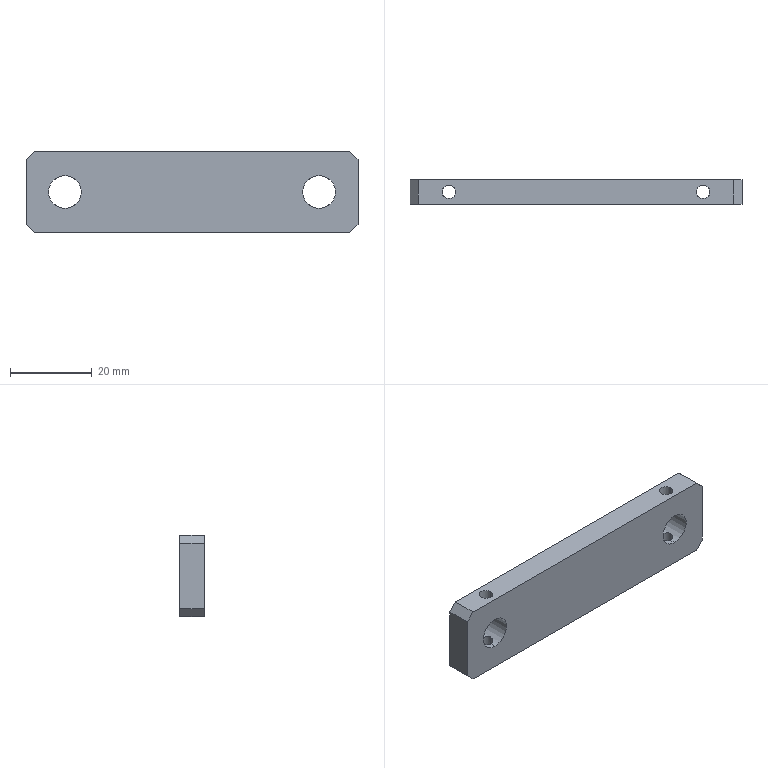Component | SolidWorks | 04LowerMaterialReceivingSwingAngleAssembly(3920)-1_H2020022-0445-1(3920)-4 | 1 solid | 22 faces | box 81 x 6 x 20 mm | volume 8861 mm3 | cylinder 12 | plane 10 | commonest cylinder face diameters 3.3 x8 8 x4 | material 45#Steel
STEP:
#1=COLOUR_RGB('',0.7922,0.8196,0.9333);
#2=FILL_AREA_STYLE_COLOUR('',#1);
#3=FILL_AREA_STYLE('',(#2));
#4=SURFACE_STYLE_FILL_AREA(#3);
#5=SURFACE_SIDE_STYLE('',(#4));
#6=SURFACE_STYLE_USAGE(.BOTH.,#5);
#7=PRESENTATION_STYLE_ASSIGNMENT((#6));
#8=CARTESIAN_POINT('',(2.377,5.032,11.175));
#9=VERTEX_POINT('',#8);
#10=CARTESIAN_POINT('',(2.442,4.967,11.189));
#11=VERTEX_POINT('',#10);
#12=CARTESIAN_POINT('',(2.377,5.032,11.175));
#13=CARTESIAN_POINT('',(2.377,5.023,11.175));
#14=CARTESIAN_POINT('',(2.379,5.015,11.176));
#15=CARTESIAN_POINT('',(2.384,5.003,11.178));
#16=CARTESIAN_POINT('',(2.386,4.999,11.178));
#17=CARTESIAN_POINT('',(2.391,4.992,11.18));
#18=CARTESIAN_POINT('',(2.393,4.989,11.181));
#19=CARTESIAN_POINT('',(2.399,4.983,11.183));
#20=CARTESIAN_POINT('',(2.403,4.98,11.184));
#21=CARTESIAN_POINT('',(2.41,4.976,11.185));
#22=CARTESIAN_POINT('',(2.413,4.974,11.186));
#23=CARTESIAN_POINT('',(2.425,4.969,11.188));
#24=CARTESIAN_POINT('',(2.434,4.967,11.189));
#25=CARTESIAN_POINT('',(2.442,4.967,11.189));
#26=B_SPLINE_CURVE_WITH_KNOTS('',3,(#12,#13,#14,#15,#16,#17,#18,#19,#20,#21,#22,#23,#24,#25),.UNSPECIFIED.,.F.,.F.,(4,2,2,2,2,2,4),(0.007825,0.008476,0.008802,0.009128,0.009454,0.00978,0.01043),.UNSPECIFIED.);
#27=EDGE_CURVE('',#9,#11,#26,.T.);
#28=ORIENTED_EDGE('',*,*,#27,.F.);
#29=CARTESIAN_POINT('',(2.377,5.032,11.425));
#30=VERTEX_POINT('',#29);
#31=CARTESIAN_POINT('',(2.377,5.032,11.425));
#32=DIRECTION('',(0.,0.,1.));
#33=VECTOR('',#32,39.37);
#34=LINE('',#31,#33);
#35=EDGE_CURVE('',#9,#30,#34,.T.);
#36=ORIENTED_EDGE('',*,*,#35,.T.);
#37=CARTESIAN_POINT('',(2.507,5.032,11.425));
#38=VERTEX_POINT('',#37);
#39=CARTESIAN_POINT('',(2.442,5.032,11.425));
#40=DIRECTION('',(0.,0.,1.));
#41=DIRECTION('',(1.,0.,0.));
#42=AXIS2_PLACEMENT_3D('',#39,#40,#41);
#43=CIRCLE('',#42,0.06496);
#44=EDGE_CURVE('',#30,#38,#43,.T.);
#45=ORIENTED_EDGE('',*,*,#44,.T.);
#46=CARTESIAN_POINT('',(2.507,5.032,11.175));
#47=VERTEX_POINT('',#46);
#48=CARTESIAN_POINT('',(2.507,5.032,11.425));
#49=DIRECTION('',(0.,0.,1.));
#50=VECTOR('',#49,39.37);
#51=LINE('',#48,#50);
#52=EDGE_CURVE('',#47,#38,#51,.T.);
#53=ORIENTED_EDGE('',*,*,#52,.F.);
#54=CARTESIAN_POINT('',(2.442,4.967,11.189));
#55=CARTESIAN_POINT('',(2.447,4.967,11.189));
#56=CARTESIAN_POINT('',(2.451,4.967,11.189));
#57=CARTESIAN_POINT('',(2.459,4.969,11.188));
#58=CARTESIAN_POINT('',(2.463,4.97,11.187));
#59=CARTESIAN_POINT('',(2.475,4.975,11.186));
#60=CARTESIAN_POINT('',(2.482,4.98,11.184));
#61=CARTESIAN_POINT('',(2.494,4.992,11.18));
#62=CARTESIAN_POINT('',(2.499,4.999,11.178));
#63=CARTESIAN_POINT('',(2.504,5.011,11.176));
#64=CARTESIAN_POINT('',(2.505,5.015,11.176));
#65=CARTESIAN_POINT('',(2.507,5.023,11.175));
#66=CARTESIAN_POINT('',(2.507,5.028,11.175));
#67=CARTESIAN_POINT('',(2.507,5.032,11.175));
#68=B_SPLINE_CURVE_WITH_KNOTS('',3,(#54,#55,#56,#57,#58,#59,#60,#61,#62,#63,#64,#65,#66,#67),.UNSPECIFIED.,.F.,.F.,(4,2,2,2,2,2,4),(0.,0.0003262,0.0006525,0.001305,0.001957,0.002284,0.00261),.UNSPECIFIED.);
#69=EDGE_CURVE('',#11,#47,#68,.T.);
#70=ORIENTED_EDGE('',*,*,#69,.F.);
#71=EDGE_LOOP('',(#28,#36,#45,#53,#70));
#72=FACE_OUTER_BOUND('',#71,.T.);
#73=CARTESIAN_POINT('',(2.442,5.032,11.425));
#74=DIRECTION('',(0.,0.,1.));
#75=DIRECTION('',(1.,0.,0.));
#76=AXIS2_PLACEMENT_3D('',#73,#74,#75);
#77=CYLINDRICAL_SURFACE('',#76,0.06496);
#78=ADVANCED_FACE('',(#72),#77,.F.);
#79=CARTESIAN_POINT('',(2.377,5.032,10.638));
#80=VERTEX_POINT('',#79);
#81=CARTESIAN_POINT('',(2.507,5.032,10.638));
#82=VERTEX_POINT('',#81);
#83=CARTESIAN_POINT('',(2.442,5.032,10.638));
#84=DIRECTION('',(0.,0.,1.));
#85=DIRECTION('',(1.,0.,0.));
#86=AXIS2_PLACEMENT_3D('',#83,#84,#85);
#87=CIRCLE('',#86,0.06496);
#88=EDGE_CURVE('',#80,#82,#87,.T.);
#89=ORIENTED_EDGE('',*,*,#88,.F.);
#90=CARTESIAN_POINT('',(2.377,5.032,10.888));
#91=VERTEX_POINT('',#90);
#92=CARTESIAN_POINT('',(2.377,5.032,11.425));
#93=DIRECTION('',(0.,0.,1.));
#94=VECTOR('',#93,39.37);
#95=LINE('',#92,#94);
#96=EDGE_CURVE('',#80,#91,#95,.T.);
#97=ORIENTED_EDGE('',*,*,#96,.T.);
#98=CARTESIAN_POINT('',(2.442,4.967,10.874));
#99=VERTEX_POINT('',#98);
#100=CARTESIAN_POINT('',(2.442,4.967,10.874));
#101=CARTESIAN_POINT('',(2.438,4.967,10.874));
#102=CARTESIAN_POINT('',(2.434,4.967,10.874));
#103=CARTESIAN_POINT('',(2.425,4.969,10.875));
#104=CARTESIAN_POINT('',(2.421,4.97,10.875));
#105=CARTESIAN_POINT('',(2.413,4.974,10.877));
#106=CARTESIAN_POINT('',(2.41,4.976,10.877));
#107=CARTESIAN_POINT('',(2.403,4.98,10.879));
#108=CARTESIAN_POINT('',(2.399,4.983,10.88));
#109=CARTESIAN_POINT('',(2.393,4.989,10.882));
#110=CARTESIAN_POINT('',(2.391,4.992,10.883));
#111=CARTESIAN_POINT('',(2.386,4.999,10.884));
#112=CARTESIAN_POINT('',(2.384,5.003,10.885));
#113=CARTESIAN_POINT('',(2.379,5.015,10.887));
#114=CARTESIAN_POINT('',(2.377,5.023,10.888));
#115=CARTESIAN_POINT('',(2.377,5.032,10.888));
#116=B_SPLINE_CURVE_WITH_KNOTS('',3,(#100,#101,#102,#103,#104,#105,#106,#107,#108,#109,#110,#111,#112,#113,#114,#115),.UNSPECIFIED.,.F.,.F.,(4,2,2,2,2,2,2,4),(0.00261,0.002935,0.003261,0.003587,0.003913,0.004239,0.004565,0.005217),.UNSPECIFIED.);
#117=EDGE_CURVE('',#99,#91,#116,.T.);
#118=ORIENTED_EDGE('',*,*,#117,.F.);
#119=CARTESIAN_POINT('',(2.507,5.032,10.888));
#120=VERTEX_POINT('',#119);
#121=CARTESIAN_POINT('',(2.507,5.032,10.888));
#122=CARTESIAN_POINT('',(2.507,5.028,10.888));
#123=CARTESIAN_POINT('',(2.507,5.023,10.888));
#124=CARTESIAN_POINT('',(2.505,5.015,10.887));
#125=CARTESIAN_POINT('',(2.504,5.011,10.886));
#126=CARTESIAN_POINT('',(2.499,4.999,10.884));
#127=CARTESIAN_POINT('',(2.494,4.992,10.883));
#128=CARTESIAN_POINT('',(2.482,4.98,10.879));
#129=CARTESIAN_POINT('',(2.475,4.975,10.877));
#130=CARTESIAN_POINT('',(2.463,4.97,10.875));
#131=CARTESIAN_POINT('',(2.459,4.969,10.875));
#132=CARTESIAN_POINT('',(2.451,4.967,10.874));
#133=CARTESIAN_POINT('',(2.447,4.967,10.874));
#134=CARTESIAN_POINT('',(2.442,4.967,10.874));
#135=B_SPLINE_CURVE_WITH_KNOTS('',3,(#121,#122,#123,#124,#125,#126,#127,#128,#129,#130,#131,#132,#133,#134),.UNSPECIFIED.,.F.,.F.,(4,2,2,2,2,2,4),(0.,0.0003262,0.0006524,0.001305,0.001957,0.002283,0.00261),.UNSPECIFIED.);
#136=EDGE_CURVE('',#120,#99,#135,.T.);
#137=ORIENTED_EDGE('',*,*,#136,.F.);
#138=CARTESIAN_POINT('',(2.507,5.032,11.425));
#139=DIRECTION('',(0.,0.,1.));
#140=VECTOR('',#139,39.37);
#141=LINE('',#138,#140);
#142=EDGE_CURVE('',#82,#120,#141,.T.);
#143=ORIENTED_EDGE('',*,*,#142,.F.);
#144=EDGE_LOOP('',(#89,#97,#118,#137,#143));
#145=FACE_OUTER_BOUND('',#144,.T.);
#146=CARTESIAN_POINT('',(2.442,5.032,11.425));
#147=DIRECTION('',(0.,0.,1.));
#148=DIRECTION('',(1.,0.,0.));
#149=AXIS2_PLACEMENT_3D('',#146,#147,#148);
#150=CYLINDRICAL_SURFACE('',#149,0.06496);
#151=ADVANCED_FACE('',(#145),#150,.F.);
#152=CARTESIAN_POINT('',(2.442,4.914,10.874));
#153=VERTEX_POINT('',#152);
#154=CARTESIAN_POINT('',(2.442,4.914,11.189));
#155=VERTEX_POINT('',#154);
#156=CARTESIAN_POINT('',(2.442,4.914,11.031));
#157=DIRECTION('',(0.,1.,0.));
#158=DIRECTION('',(0.,0.,1.));
#159=AXIS2_PLACEMENT_3D('',#156,#157,#158);
#160=CIRCLE('',#159,0.1575);
#161=EDGE_CURVE('',#153,#155,#160,.T.);
#162=ORIENTED_EDGE('',*,*,#161,.F.);
#163=CARTESIAN_POINT('',(2.442,4.914,10.874));
#164=DIRECTION('',(0.,1.,0.));
#165=VECTOR('',#164,39.37);
#166=LINE('',#163,#165);
#167=EDGE_CURVE('',#153,#99,#166,.T.);
#168=ORIENTED_EDGE('',*,*,#167,.T.);
#169=ORIENTED_EDGE('',*,*,#117,.T.);
#170=CARTESIAN_POINT('',(2.442,5.097,10.874));
#171=VERTEX_POINT('',#170);
#172=CARTESIAN_POINT('',(2.377,5.032,10.888));
#173=CARTESIAN_POINT('',(2.377,5.036,10.888));
#174=CARTESIAN_POINT('',(2.378,5.041,10.888));
#175=CARTESIAN_POINT('',(2.38,5.049,10.887));
#176=CARTESIAN_POINT('',(2.381,5.053,10.886));
#177=CARTESIAN_POINT('',(2.386,5.065,10.884));
#178=CARTESIAN_POINT('',(2.39,5.072,10.883));
#179=CARTESIAN_POINT('',(2.399,5.081,10.88));
#180=CARTESIAN_POINT('',(2.403,5.084,10.879));
#181=CARTESIAN_POINT('',(2.41,5.088,10.877));
#182=CARTESIAN_POINT('',(2.413,5.09,10.877));
#183=CARTESIAN_POINT('',(2.421,5.094,10.875));
#184=CARTESIAN_POINT('',(2.425,5.095,10.875));
#185=CARTESIAN_POINT('',(2.434,5.097,10.874));
#186=CARTESIAN_POINT('',(2.438,5.097,10.874));
#187=CARTESIAN_POINT('',(2.442,5.097,10.874));
#188=B_SPLINE_CURVE_WITH_KNOTS('',3,(#172,#173,#174,#175,#176,#177,#178,#179,#180,#181,#182,#183,#184,#185,#186,#187),.UNSPECIFIED.,.F.,.F.,(4,2,2,2,2,2,2,4),(0.005217,0.005543,0.005869,0.006521,0.006847,0.007172,0.007498,0.007824),.UNSPECIFIED.);
#189=EDGE_CURVE('',#91,#171,#188,.T.);
#190=ORIENTED_EDGE('',*,*,#189,.T.);
#191=CARTESIAN_POINT('',(2.442,5.15,10.874));
#192=VERTEX_POINT('',#191);
#193=CARTESIAN_POINT('',(2.442,4.914,10.874));
#194=DIRECTION('',(0.,1.,0.));
#195=VECTOR('',#194,39.37);
#196=LINE('',#193,#195);
#197=EDGE_CURVE('',#171,#192,#196,.T.);
#198=ORIENTED_EDGE('',*,*,#197,.T.);
#199=CARTESIAN_POINT('',(2.442,5.15,11.189));
#200=VERTEX_POINT('',#199);
#201=CARTESIAN_POINT('',(2.442,5.15,11.031));
#202=DIRECTION('',(0.,1.,0.));
#203=DIRECTION('',(0.,0.,1.));
#204=AXIS2_PLACEMENT_3D('',#201,#202,#203);
#205=CIRCLE('',#204,0.1575);
#206=EDGE_CURVE('',#192,#200,#205,.T.);
#207=ORIENTED_EDGE('',*,*,#206,.T.);
#208=CARTESIAN_POINT('',(2.442,5.097,11.189));
#209=VERTEX_POINT('',#208);
#210=CARTESIAN_POINT('',(2.442,4.914,11.189));
#211=DIRECTION('',(0.,1.,0.));
#212=VECTOR('',#211,39.37);
#213=LINE('',#210,#212);
#214=EDGE_CURVE('',#209,#200,#213,.T.);
#215=ORIENTED_EDGE('',*,*,#214,.F.);
#216=CARTESIAN_POINT('',(2.442,5.097,11.189));
#217=CARTESIAN_POINT('',(2.438,5.097,11.189));
#218=CARTESIAN_POINT('',(2.434,5.097,11.189));
#219=CARTESIAN_POINT('',(2.425,5.095,11.188));
#220=CARTESIAN_POINT('',(2.421,5.094,11.187));
#221=CARTESIAN_POINT('',(2.409,5.089,11.186));
#222=CARTESIAN_POINT('',(2.402,5.084,11.184));
#223=CARTESIAN_POINT('',(2.393,5.075,11.181));
#224=CARTESIAN_POINT('',(2.391,5.072,11.18));
#225=CARTESIAN_POINT('',(2.386,5.065,11.178));
#226=CARTESIAN_POINT('',(2.384,5.061,11.178));
#227=CARTESIAN_POINT('',(2.381,5.053,11.176));
#228=CARTESIAN_POINT('',(2.38,5.049,11.176));
#229=CARTESIAN_POINT('',(2.378,5.041,11.175));
#230=CARTESIAN_POINT('',(2.377,5.036,11.175));
#231=CARTESIAN_POINT('',(2.377,5.032,11.175));
#232=B_SPLINE_CURVE_WITH_KNOTS('',3,(#216,#217,#218,#219,#220,#221,#222,#223,#224,#225,#226,#227,#228,#229,#230,#231),.UNSPECIFIED.,.F.,.F.,(4,2,2,2,2,2,2,4),(0.005218,0.005543,0.005869,0.006521,0.006847,0.007173,0.007499,0.007825),.UNSPECIFIED.);
#233=EDGE_CURVE('',#209,#9,#232,.T.);
#234=ORIENTED_EDGE('',*,*,#233,.T.);
#235=ORIENTED_EDGE('',*,*,#27,.T.);
#236=CARTESIAN_POINT('',(2.442,4.914,11.189));
#237=DIRECTION('',(0.,1.,0.));
#238=VECTOR('',#237,39.37);
#239=LINE('',#236,#238);
#240=EDGE_CURVE('',#155,#11,#239,.T.);
#241=ORIENTED_EDGE('',*,*,#240,.F.);
#242=EDGE_LOOP('',(#162,#168,#169,#190,#198,#207,#215,#234,#235,#241));
#243=FACE_OUTER_BOUND('',#242,.T.);
#244=CARTESIAN_POINT('',(2.442,4.914,11.031));
#245=DIRECTION('',(0.,1.,0.));
#246=DIRECTION('',(0.,0.,1.));
#247=AXIS2_PLACEMENT_3D('',#244,#245,#246);
#248=CYLINDRICAL_SURFACE('',#247,0.1575);
#249=ADVANCED_FACE('',(#243),#248,.F.);
#250=CARTESIAN_POINT('',(-0.06355,5.032,11.175));
#251=VERTEX_POINT('',#250);
#252=CARTESIAN_POINT('',(0.001409,4.967,11.189));
#253=VERTEX_POINT('',#252);
#254=CARTESIAN_POINT('',(-0.06355,5.032,11.175));
#255=CARTESIAN_POINT('',(-0.06355,5.023,11.175));
#256=CARTESIAN_POINT('',(-0.06181,5.015,11.176));
#257=CARTESIAN_POINT('',(-0.05691,5.003,11.178));
#258=CARTESIAN_POINT('',(-0.05488,4.999,11.178));
#259=CARTESIAN_POINT('',(-0.05018,4.992,11.18));
#260=CARTESIAN_POINT('',(-0.04752,4.989,11.181));
#261=CARTESIAN_POINT('',(-0.04156,4.983,11.183));
#262=CARTESIAN_POINT('',(-0.03828,4.98,11.184));
#263=CARTESIAN_POINT('',(-0.03131,4.976,11.185));
#264=CARTESIAN_POINT('',(-0.0276,4.974,11.186));
#265=CARTESIAN_POINT('',(-0.01571,4.969,11.188));
#266=CARTESIAN_POINT('',(-0.007272,4.967,11.189));
#267=CARTESIAN_POINT('',(0.001409,4.967,11.189));
#268=B_SPLINE_CURVE_WITH_KNOTS('',3,(#254,#255,#256,#257,#258,#259,#260,#261,#262,#263,#264,#265,#266,#267),.UNSPECIFIED.,.F.,.F.,(4,2,2,2,2,2,4),(0.007825,0.008476,0.008802,0.009128,0.009454,0.00978,0.01043),.UNSPECIFIED.);
#269=EDGE_CURVE('',#251,#253,#268,.T.);
#270=ORIENTED_EDGE('',*,*,#269,.F.);
#271=CARTESIAN_POINT('',(-0.06355,5.032,11.425));
#272=VERTEX_POINT('',#271);
#273=CARTESIAN_POINT('',(-0.06355,5.032,11.425));
#274=DIRECTION('',(0.,0.,1.));
#275=VECTOR('',#274,39.37);
#276=LINE('',#273,#275);
#277=EDGE_CURVE('',#251,#272,#276,.T.);
#278=ORIENTED_EDGE('',*,*,#277,.T.);
#279=CARTESIAN_POINT('',(0.06637,5.032,11.425));
#280=VERTEX_POINT('',#279);
#281=CARTESIAN_POINT('',(0.001409,5.032,11.425));
#282=DIRECTION('',(0.,0.,1.));
#283=DIRECTION('',(1.,0.,0.));
#284=AXIS2_PLACEMENT_3D('',#281,#282,#283);
#285=CIRCLE('',#284,0.06496);
#286=EDGE_CURVE('',#272,#280,#285,.T.);
#287=ORIENTED_EDGE('',*,*,#286,.T.);
#288=CARTESIAN_POINT('',(0.06637,5.032,11.175));
#289=VERTEX_POINT('',#288);
#290=CARTESIAN_POINT('',(0.06637,5.032,11.425));
#291=DIRECTION('',(0.,0.,1.));
#292=VECTOR('',#291,39.37);
#293=LINE('',#290,#292);
#294=EDGE_CURVE('',#289,#280,#293,.T.);
#295=ORIENTED_EDGE('',*,*,#294,.F.);
#296=CARTESIAN_POINT('',(0.001409,4.967,11.189));
#297=CARTESIAN_POINT('',(0.005755,4.967,11.189));
#298=CARTESIAN_POINT('',(0.01002,4.967,11.189));
#299=CARTESIAN_POINT('',(0.01839,4.969,11.188));
#300=CARTESIAN_POINT('',(0.02255,4.97,11.187));
#301=CARTESIAN_POINT('',(0.03433,4.975,11.186));
#302=CARTESIAN_POINT('',(0.04147,4.98,11.184));
#303=CARTESIAN_POINT('',(0.05331,4.992,11.18));
#304=CARTESIAN_POINT('',(0.05811,4.999,11.178));
#305=CARTESIAN_POINT('',(0.06299,5.011,11.176));
#306=CARTESIAN_POINT('',(0.06426,5.015,11.176));
#307=CARTESIAN_POINT('',(0.06595,5.023,11.175));
#308=CARTESIAN_POINT('',(0.06637,5.028,11.175));
#309=CARTESIAN_POINT('',(0.06637,5.032,11.175));
#310=B_SPLINE_CURVE_WITH_KNOTS('',3,(#296,#297,#298,#299,#300,#301,#302,#303,#304,#305,#306,#307,#308,#309),.UNSPECIFIED.,.F.,.F.,(4,2,2,2,2,2,4),(0.,0.0003262,0.0006525,0.001305,0.001957,0.002284,0.00261),.UNSPECIFIED.);
#311=EDGE_CURVE('',#253,#289,#310,.T.);
#312=ORIENTED_EDGE('',*,*,#311,.F.);
#313=EDGE_LOOP('',(#270,#278,#287,#295,#312));
#314=FACE_OUTER_BOUND('',#313,.T.);
#315=CARTESIAN_POINT('',(0.001409,5.032,11.425));
#316=DIRECTION('',(0.,0.,1.));
#317=DIRECTION('',(1.,0.,0.));
#318=AXIS2_PLACEMENT_3D('',#315,#316,#317);
#319=CYLINDRICAL_SURFACE('',#318,0.06496);
#320=ADVANCED_FACE('',(#314),#319,.F.);
#321=CARTESIAN_POINT('',(-0.06355,5.032,10.638));
#322=VERTEX_POINT('',#321);
#323=CARTESIAN_POINT('',(0.06637,5.032,10.638));
#324=VERTEX_POINT('',#323);
#325=CARTESIAN_POINT('',(0.001409,5.032,10.638));
#326=DIRECTION('',(0.,0.,1.));
#327=DIRECTION('',(1.,0.,0.));
#328=AXIS2_PLACEMENT_3D('',#325,#326,#327);
#329=CIRCLE('',#328,0.06496);
#330=EDGE_CURVE('',#322,#324,#329,.T.);
#331=ORIENTED_EDGE('',*,*,#330,.F.);
#332=CARTESIAN_POINT('',(-0.06355,5.032,10.888));
#333=VERTEX_POINT('',#332);
#334=CARTESIAN_POINT('',(-0.06355,5.032,11.425));
#335=DIRECTION('',(0.,0.,1.));
#336=VECTOR('',#335,39.37);
#337=LINE('',#334,#336);
#338=EDGE_CURVE('',#322,#333,#337,.T.);
#339=ORIENTED_EDGE('',*,*,#338,.T.);
#340=CARTESIAN_POINT('',(0.001409,4.967,10.874));
#341=VERTEX_POINT('',#340);
#342=CARTESIAN_POINT('',(0.001409,4.967,10.874));
#343=CARTESIAN_POINT('',(-0.002885,4.967,10.874));
#344=CARTESIAN_POINT('',(-0.007238,4.967,10.874));
#345=CARTESIAN_POINT('',(-0.01561,4.969,10.875));
#346=CARTESIAN_POINT('',(-0.0197,4.97,10.875));
#347=CARTESIAN_POINT('',(-0.02761,4.974,10.877));
#348=CARTESIAN_POINT('',(-0.03133,4.976,10.877));
#349=CARTESIAN_POINT('',(-0.03832,4.98,10.879));
#350=CARTESIAN_POINT('',(-0.04162,4.983,10.88));
#351=CARTESIAN_POINT('',(-0.04755,4.989,10.882));
#352=CARTESIAN_POINT('',(-0.05021,4.992,10.883));
#353=CARTESIAN_POINT('',(-0.05491,4.999,10.884));
#354=CARTESIAN_POINT('',(-0.05693,5.003,10.885));
#355=CARTESIAN_POINT('',(-0.0618,5.015,10.887));
#356=CARTESIAN_POINT('',(-0.06355,5.023,10.888));
#357=CARTESIAN_POINT('',(-0.06355,5.032,10.888));
#358=B_SPLINE_CURVE_WITH_KNOTS('',3,(#342,#343,#344,#345,#346,#347,#348,#349,#350,#351,#352,#353,#354,#355,#356,#357),.UNSPECIFIED.,.F.,.F.,(4,2,2,2,2,2,2,4),(0.00261,0.002935,0.003261,0.003587,0.003913,0.004239,0.004565,0.005217),.UNSPECIFIED.);
#359=EDGE_CURVE('',#341,#333,#358,.T.);
#360=ORIENTED_EDGE('',*,*,#359,.F.);
#361=CARTESIAN_POINT('',(0.06637,5.032,10.888));
#362=VERTEX_POINT('',#361);
#363=CARTESIAN_POINT('',(0.06637,5.032,10.888));
#364=CARTESIAN_POINT('',(0.06637,5.028,10.888));
#365=CARTESIAN_POINT('',(0.06594,5.023,10.888));
#366=CARTESIAN_POINT('',(0.06426,5.015,10.887));
#367=CARTESIAN_POINT('',(0.06298,5.011,10.886));
#368=CARTESIAN_POINT('',(0.05807,4.999,10.884));
#369=CARTESIAN_POINT('',(0.05326,4.992,10.883));
#370=CARTESIAN_POINT('',(0.0414,4.98,10.879));
#371=CARTESIAN_POINT('',(0.03424,4.975,10.877));
#372=CARTESIAN_POINT('',(0.02252,4.97,10.875));
#373=CARTESIAN_POINT('',(0.01837,4.969,10.875));
#374=CARTESIAN_POINT('',(0.009958,4.967,10.874));
#375=CARTESIAN_POINT('',(0.005706,4.967,10.874));
#376=CARTESIAN_POINT('',(0.001409,4.967,10.874));
#377=B_SPLINE_CURVE_WITH_KNOTS('',3,(#363,#364,#365,#366,#367,#368,#369,#370,#371,#372,#373,#374,#375,#376),.UNSPECIFIED.,.F.,.F.,(4,2,2,2,2,2,4),(0.,0.0003262,0.0006524,0.001305,0.001957,0.002283,0.00261),.UNSPECIFIED.);
#378=EDGE_CURVE('',#362,#341,#377,.T.);
#379=ORIENTED_EDGE('',*,*,#378,.F.);
#380=CARTESIAN_POINT('',(0.06637,5.032,11.425));
#381=DIRECTION('',(0.,0.,1.));
#382=VECTOR('',#381,39.37);
#383=LINE('',#380,#382);
#384=EDGE_CURVE('',#324,#362,#383,.T.);
#385=ORIENTED_EDGE('',*,*,#384,.F.);
#386=EDGE_LOOP('',(#331,#339,#360,#379,#385));
#387=FACE_OUTER_BOUND('',#386,.T.);
#388=CARTESIAN_POINT('',(0.001409,5.032,11.425));
#389=DIRECTION('',(0.,0.,1.));
#390=DIRECTION('',(1.,0.,0.));
#391=AXIS2_PLACEMENT_3D('',#388,#389,#390);
#392=CYLINDRICAL_SURFACE('',#391,0.06496);
#393=ADVANCED_FACE('',(#387),#392,.F.);
#394=CARTESIAN_POINT('',(0.001409,4.914,10.874));
#395=VERTEX_POINT('',#394);
#396=CARTESIAN_POINT('',(0.001409,4.914,11.189));
#397=VERTEX_POINT('',#396);
#398=CARTESIAN_POINT('',(0.001409,4.914,11.031));
#399=DIRECTION('',(0.,1.,0.));
#400=DIRECTION('',(0.,0.,1.));
#401=AXIS2_PLACEMENT_3D('',#398,#399,#400);
#402=CIRCLE('',#401,0.1575);
#403=EDGE_CURVE('',#395,#397,#402,.T.);
#404=ORIENTED_EDGE('',*,*,#403,.F.);
#405=CARTESIAN_POINT('',(0.001409,4.914,10.874));
#406=DIRECTION('',(0.,1.,0.));
#407=VECTOR('',#406,39.37);
#408=LINE('',#405,#407);
#409=EDGE_CURVE('',#395,#341,#408,.T.);
#410=ORIENTED_EDGE('',*,*,#409,.T.);
#411=ORIENTED_EDGE('',*,*,#359,.T.);
#412=CARTESIAN_POINT('',(0.001409,5.097,10.874));
#413=VERTEX_POINT('',#412);
#414=CARTESIAN_POINT('',(-0.06355,5.032,10.888));
#415=CARTESIAN_POINT('',(-0.06355,5.036,10.888));
#416=CARTESIAN_POINT('',(-0.06312,5.041,10.888));
#417=CARTESIAN_POINT('',(-0.06143,5.049,10.887));
#418=CARTESIAN_POINT('',(-0.06018,5.053,10.886));
#419=CARTESIAN_POINT('',(-0.05526,5.065,10.884));
#420=CARTESIAN_POINT('',(-0.05049,5.072,10.883));
#421=CARTESIAN_POINT('',(-0.04152,5.081,10.88));
#422=CARTESIAN_POINT('',(-0.03828,5.084,10.879));
#423=CARTESIAN_POINT('',(-0.03131,5.088,10.877));
#424=CARTESIAN_POINT('',(-0.02752,5.09,10.877));
#425=CARTESIAN_POINT('',(-0.01967,5.094,10.875));
#426=CARTESIAN_POINT('',(-0.01562,5.095,10.875));
#427=CARTESIAN_POINT('',(-0.007229,5.097,10.874));
#428=CARTESIAN_POINT('',(-0.002873,5.097,10.874));
#429=CARTESIAN_POINT('',(0.001409,5.097,10.874));
#430=B_SPLINE_CURVE_WITH_KNOTS('',3,(#414,#415,#416,#417,#418,#419,#420,#421,#422,#423,#424,#425,#426,#427,#428,#429),.UNSPECIFIED.,.F.,.F.,(4,2,2,2,2,2,2,4),(0.005217,0.005543,0.005869,0.006521,0.006847,0.007172,0.007498,0.007824),.UNSPECIFIED.);
#431=EDGE_CURVE('',#333,#413,#430,.T.);
#432=ORIENTED_EDGE('',*,*,#431,.T.);
#433=CARTESIAN_POINT('',(0.001409,5.15,10.874));
#434=VERTEX_POINT('',#433);
#435=CARTESIAN_POINT('',(0.001409,4.914,10.874));
#436=DIRECTION('',(0.,1.,0.));
#437=VECTOR('',#436,39.37);
#438=LINE('',#435,#437);
#439=EDGE_CURVE('',#413,#434,#438,.T.);
#440=ORIENTED_EDGE('',*,*,#439,.T.);
#441=CARTESIAN_POINT('',(0.001409,5.15,11.189));
#442=VERTEX_POINT('',#441);
#443=CARTESIAN_POINT('',(0.001409,5.15,11.031));
#444=DIRECTION('',(0.,1.,0.));
#445=DIRECTION('',(0.,0.,1.));
#446=AXIS2_PLACEMENT_3D('',#443,#444,#445);
#447=CIRCLE('',#446,0.1575);
#448=EDGE_CURVE('',#434,#442,#447,.T.);
#449=ORIENTED_EDGE('',*,*,#448,.T.);
#450=CARTESIAN_POINT('',(0.001409,5.097,11.189));
#451=VERTEX_POINT('',#450);
#452=CARTESIAN_POINT('',(0.001409,4.914,11.189));
#453=DIRECTION('',(0.,1.,0.));
#454=VECTOR('',#453,39.37);
#455=LINE('',#452,#454);
#456=EDGE_CURVE('',#451,#442,#455,.T.);
#457=ORIENTED_EDGE('',*,*,#456,.F.);
#458=CARTESIAN_POINT('',(0.001409,5.097,11.189));
#459=CARTESIAN_POINT('',(-0.002868,5.097,11.189));
#460=CARTESIAN_POINT('',(-0.007207,5.097,11.189));
#461=CARTESIAN_POINT('',(-0.01562,5.095,11.188));
#462=CARTESIAN_POINT('',(-0.01969,5.094,11.187));
#463=CARTESIAN_POINT('',(-0.03149,5.089,11.186));
#464=CARTESIAN_POINT('',(-0.03859,5.084,11.184));
#465=CARTESIAN_POINT('',(-0.04756,5.075,11.181));
#466=CARTESIAN_POINT('',(-0.05021,5.072,11.18));
#467=CARTESIAN_POINT('',(-0.05489,5.065,11.178));
#468=CARTESIAN_POINT('',(-0.05692,5.061,11.178));
#469=CARTESIAN_POINT('',(-0.06019,5.053,11.176));
#470=CARTESIAN_POINT('',(-0.06143,5.049,11.176));
#471=CARTESIAN_POINT('',(-0.06312,5.041,11.175));
#472=CARTESIAN_POINT('',(-0.06355,5.036,11.175));
#473=CARTESIAN_POINT('',(-0.06355,5.032,11.175));
#474=B_SPLINE_CURVE_WITH_KNOTS('',3,(#458,#459,#460,#461,#462,#463,#464,#465,#466,#467,#468,#469,#470,#471,#472,#473),.UNSPECIFIED.,.F.,.F.,(4,2,2,2,2,2,2,4),(0.005218,0.005543,0.005869,0.006521,0.006847,0.007173,0.007499,0.007825),.UNSPECIFIED.);
#475=EDGE_CURVE('',#451,#251,#474,.T.);
#476=ORIENTED_EDGE('',*,*,#475,.T.);
#477=ORIENTED_EDGE('',*,*,#269,.T.);
#478=CARTESIAN_POINT('',(0.001409,4.914,11.189));
#479=DIRECTION('',(0.,1.,0.));
#480=VECTOR('',#479,39.37);
#481=LINE('',#478,#480);
#482=EDGE_CURVE('',#397,#253,#481,.T.);
#483=ORIENTED_EDGE('',*,*,#482,.F.);
#484=EDGE_LOOP('',(#404,#410,#411,#432,#440,#449,#457,#476,#477,#483));
#485=FACE_OUTER_BOUND('',#484,.T.);
#486=CARTESIAN_POINT('',(0.001409,4.914,11.031));
#487=DIRECTION('',(0.,1.,0.));
#488=DIRECTION('',(0.,0.,1.));
#489=AXIS2_PLACEMENT_3D('',#486,#487,#488);
#490=CYLINDRICAL_SURFACE('',#489,0.1575);
#491=ADVANCED_FACE('',(#485),#490,.F.);
#492=CARTESIAN_POINT('',(-0.3726,5.15,10.716));
#493=VERTEX_POINT('',#492);
#494=CARTESIAN_POINT('',(-0.3726,5.15,11.346));
#495=VERTEX_POINT('',#494);
#496=CARTESIAN_POINT('',(-0.3726,5.15,10.638));
#497=DIRECTION('',(0.,0.,1.));
#498=VECTOR('',#497,39.37);
#499=LINE('',#496,#498);
#500=EDGE_CURVE('',#493,#495,#499,.T.);
#501=ORIENTED_EDGE('',*,*,#500,.F.);
#502=CARTESIAN_POINT('',(-0.3726,4.914,10.716));
#503=VERTEX_POINT('',#502);
#504=CARTESIAN_POINT('',(-0.3726,5.15,10.716));
#505=DIRECTION('',(0.,-1.,0.));
#506=VECTOR('',#505,39.37);
#507=LINE('',#504,#506);
#508=EDGE_CURVE('',#493,#503,#507,.T.);
#509=ORIENTED_EDGE('',*,*,#508,.T.);
#510=CARTESIAN_POINT('',(-0.3726,4.914,11.346));
#511=VERTEX_POINT('',#510);
#512=CARTESIAN_POINT('',(-0.3726,4.914,10.638));
#513=DIRECTION('',(0.,0.,1.));
#514=VECTOR('',#513,39.37);
#515=LINE('',#512,#514);
#516=EDGE_CURVE('',#503,#511,#515,.T.);
#517=ORIENTED_EDGE('',*,*,#516,.T.);
#518=CARTESIAN_POINT('',(-0.3726,5.15,11.346));
#519=DIRECTION('',(0.,1.,0.));
#520=VECTOR('',#519,39.37);
#521=LINE('',#518,#520);
#522=EDGE_CURVE('',#511,#495,#521,.T.);
#523=ORIENTED_EDGE('',*,*,#522,.T.);
#524=EDGE_LOOP('',(#501,#509,#517,#523));
#525=FACE_OUTER_BOUND('',#524,.T.);
#526=CARTESIAN_POINT('',(-0.3726,5.15,10.638));
#527=DIRECTION('',(1.,0.,-0.));
#528=DIRECTION('',(-0.,0.,-1.));
#529=AXIS2_PLACEMENT_3D('',#526,#527,#528);
#530=PLANE('',#529);
#531=ADVANCED_FACE('',(#525),#530,.F.);
#532=CARTESIAN_POINT('',(2.442,5.032,11.425));
#533=DIRECTION('',(0.,0.,1.));
#534=DIRECTION('',(1.,0.,0.));
#535=AXIS2_PLACEMENT_3D('',#532,#533,#534);
#536=CIRCLE('',#535,0.06496);
#537=EDGE_CURVE('',#38,#30,#536,.T.);
#538=ORIENTED_EDGE('',*,*,#537,.F.);
#539=ORIENTED_EDGE('',*,*,#44,.F.);
#540=EDGE_LOOP('',(#538,#539));
#541=FACE_BOUND('',#540,.T.);
#542=CARTESIAN_POINT('',(0.001409,5.032,11.425));
#543=DIRECTION('',(0.,0.,1.));
#544=DIRECTION('',(1.,0.,0.));
#545=AXIS2_PLACEMENT_3D('',#542,#543,#544);
#546=CIRCLE('',#545,0.06496);
#547=EDGE_CURVE('',#280,#272,#546,.T.);
#548=ORIENTED_EDGE('',*,*,#547,.F.);
#549=ORIENTED_EDGE('',*,*,#286,.F.);
#550=EDGE_LOOP('',(#548,#549));
#551=FACE_BOUND('',#550,.T.);
#552=CARTESIAN_POINT('',(-0.2939,5.15,11.425));
#553=VERTEX_POINT('',#552);
#554=CARTESIAN_POINT('',(2.738,5.15,11.425));
#555=VERTEX_POINT('',#554);
#556=CARTESIAN_POINT('',(-0.3726,5.15,11.425));
#557=DIRECTION('',(1.,0.,0.));
#558=VECTOR('',#557,39.37);
#559=LINE('',#556,#558);
#560=EDGE_CURVE('',#553,#555,#559,.T.);
#561=ORIENTED_EDGE('',*,*,#560,.F.);
#562=CARTESIAN_POINT('',(-0.2939,4.914,11.425));
#563=VERTEX_POINT('',#562);
#564=CARTESIAN_POINT('',(-0.2939,5.15,11.425));
#565=DIRECTION('',(0.,-1.,0.));
#566=VECTOR('',#565,39.37);
#567=LINE('',#564,#566);
#568=EDGE_CURVE('',#553,#563,#567,.T.);
#569=ORIENTED_EDGE('',*,*,#568,.T.);
#570=CARTESIAN_POINT('',(2.738,4.914,11.425));
#571=VERTEX_POINT('',#570);
#572=CARTESIAN_POINT('',(-0.3726,4.914,11.425));
#573=DIRECTION('',(1.,0.,0.));
#574=VECTOR('',#573,39.37);
#575=LINE('',#572,#574);
#576=EDGE_CURVE('',#563,#571,#575,.T.);
#577=ORIENTED_EDGE('',*,*,#576,.T.);
#578=CARTESIAN_POINT('',(2.738,5.15,11.425));
#579=DIRECTION('',(0.,1.,0.));
#580=VECTOR('',#579,39.37);
#581=LINE('',#578,#580);
#582=EDGE_CURVE('',#571,#555,#581,.T.);
#583=ORIENTED_EDGE('',*,*,#582,.T.);
#584=EDGE_LOOP('',(#561,#569,#577,#583));
#585=FACE_OUTER_BOUND('',#584,.T.);
#586=CARTESIAN_POINT('',(-0.3726,5.15,11.425));
#587=DIRECTION('',(0.,0.,-1.));
#588=DIRECTION('',(-1.,0.,0.));
#589=AXIS2_PLACEMENT_3D('',#586,#587,#588);
#590=PLANE('',#589);
#591=ADVANCED_FACE('',(#541,#551,#585),#590,.F.);
#592=CARTESIAN_POINT('',(2.816,4.914,11.346));
#593=VERTEX_POINT('',#592);
#594=CARTESIAN_POINT('',(2.816,4.914,10.716));
#595=VERTEX_POINT('',#594);
#596=CARTESIAN_POINT('',(2.816,4.914,10.638));
#597=DIRECTION('',(0.,0.,-1.));
#598=VECTOR('',#597,39.37);
#599=LINE('',#596,#598);
#600=EDGE_CURVE('',#593,#595,#599,.T.);
#601=ORIENTED_EDGE('',*,*,#600,.T.);
#602=CARTESIAN_POINT('',(2.816,5.15,10.716));
#603=VERTEX_POINT('',#602);
#604=CARTESIAN_POINT('',(2.816,5.15,10.716));
#605=DIRECTION('',(0.,1.,0.));
#606=VECTOR('',#605,39.37);
#607=LINE('',#604,#606);
#608=EDGE_CURVE('',#595,#603,#607,.T.);
#609=ORIENTED_EDGE('',*,*,#608,.T.);
#610=CARTESIAN_POINT('',(2.816,5.15,11.346));
#611=VERTEX_POINT('',#610);
#612=CARTESIAN_POINT('',(2.816,5.15,10.638));
#613=DIRECTION('',(0.,0.,-1.));
#614=VECTOR('',#613,39.37);
#615=LINE('',#612,#614);
#616=EDGE_CURVE('',#611,#603,#615,.T.);
#617=ORIENTED_EDGE('',*,*,#616,.F.);
#618=CARTESIAN_POINT('',(2.816,5.15,11.346));
#619=DIRECTION('',(0.,-1.,0.));
#620=VECTOR('',#619,39.37);
#621=LINE('',#618,#620);
#622=EDGE_CURVE('',#611,#593,#621,.T.);
#623=ORIENTED_EDGE('',*,*,#622,.T.);
#624=EDGE_LOOP('',(#601,#609,#617,#623));
#625=FACE_OUTER_BOUND('',#624,.T.);
#626=CARTESIAN_POINT('',(2.816,5.15,10.638));
#627=DIRECTION('',(-1.,0.,0.));
#628=DIRECTION('',(0.,0.,1.));
#629=AXIS2_PLACEMENT_3D('',#626,#627,#628);
#630=PLANE('',#629);
#631=ADVANCED_FACE('',(#625),#630,.F.);
#632=CARTESIAN_POINT('',(2.442,5.032,10.638));
#633=DIRECTION('',(0.,0.,1.));
#634=DIRECTION('',(1.,0.,0.));
#635=AXIS2_PLACEMENT_3D('',#632,#633,#634);
#636=CIRCLE('',#635,0.06496);
#637=EDGE_CURVE('',#82,#80,#636,.T.);
#638=ORIENTED_EDGE('',*,*,#637,.T.);
#639=ORIENTED_EDGE('',*,*,#88,.T.);
#640=EDGE_LOOP('',(#638,#639));
#641=FACE_BOUND('',#640,.T.);
#642=CARTESIAN_POINT('',(0.001409,5.032,10.638));
#643=DIRECTION('',(0.,0.,1.));
#644=DIRECTION('',(1.,0.,0.));
#645=AXIS2_PLACEMENT_3D('',#642,#643,#644);
#646=CIRCLE('',#645,0.06496);
#647=EDGE_CURVE('',#324,#322,#646,.T.);
#648=ORIENTED_EDGE('',*,*,#647,.T.);
#649=ORIENTED_EDGE('',*,*,#330,.T.);
#650=EDGE_LOOP('',(#648,#649));
#651=FACE_BOUND('',#650,.T.);
#652=CARTESIAN_POINT('',(2.738,4.914,10.638));
#653=VERTEX_POINT('',#652);
#654=CARTESIAN_POINT('',(-0.2939,4.914,10.638));
#655=VERTEX_POINT('',#654);
#656=CARTESIAN_POINT('',(-0.3726,4.914,10.638));
#657=DIRECTION('',(-1.,0.,0.));
#658=VECTOR('',#657,39.37);
#659=LINE('',#656,#658);
#660=EDGE_CURVE('',#653,#655,#659,.T.);
#661=ORIENTED_EDGE('',*,*,#660,.T.);
#662=CARTESIAN_POINT('',(-0.2939,5.15,10.638));
#663=VERTEX_POINT('',#662);
#664=CARTESIAN_POINT('',(-0.2939,5.15,10.638));
#665=DIRECTION('',(0.,1.,0.));
#666=VECTOR('',#665,39.37);
#667=LINE('',#664,#666);
#668=EDGE_CURVE('',#655,#663,#667,.T.);
#669=ORIENTED_EDGE('',*,*,#668,.T.);
#670=CARTESIAN_POINT('',(2.738,5.15,10.638));
#671=VERTEX_POINT('',#670);
#672=CARTESIAN_POINT('',(-0.3726,5.15,10.638));
#673=DIRECTION('',(-1.,0.,0.));
#674=VECTOR('',#673,39.37);
#675=LINE('',#672,#674);
#676=EDGE_CURVE('',#671,#663,#675,.T.);
#677=ORIENTED_EDGE('',*,*,#676,.F.);
#678=CARTESIAN_POINT('',(2.738,5.15,10.638));
#679=DIRECTION('',(0.,-1.,0.));
#680=VECTOR('',#679,39.37);
#681=LINE('',#678,#680);
#682=EDGE_CURVE('',#671,#653,#681,.T.);
#683=ORIENTED_EDGE('',*,*,#682,.T.);
#684=EDGE_LOOP('',(#661,#669,#677,#683));
#685=FACE_OUTER_BOUND('',#684,.T.);
#686=CARTESIAN_POINT('',(-0.3726,5.15,10.638));
#687=DIRECTION('',(0.,0.,1.));
#688=DIRECTION('',(1.,0.,0.));
#689=AXIS2_PLACEMENT_3D('',#686,#687,#688);
#690=PLANE('',#689);
#691=ADVANCED_FACE('',(#641,#651,#685),#690,.F.);
#692=CARTESIAN_POINT('',(2.442,5.15,11.031));
#693=DIRECTION('',(0.,1.,0.));
#694=DIRECTION('',(0.,0.,1.));
#695=AXIS2_PLACEMENT_3D('',#692,#693,#694);
#696=CIRCLE('',#695,0.1575);
#697=EDGE_CURVE('',#200,#192,#696,.T.);
#698=ORIENTED_EDGE('',*,*,#697,.F.);
#699=ORIENTED_EDGE('',*,*,#206,.F.);
#700=EDGE_LOOP('',(#698,#699));
#701=FACE_BOUND('',#700,.T.);
#702=CARTESIAN_POINT('',(0.001409,5.15,11.031));
#703=DIRECTION('',(0.,1.,0.));
#704=DIRECTION('',(0.,0.,1.));
#705=AXIS2_PLACEMENT_3D('',#702,#703,#704);
#706=CIRCLE('',#705,0.1575);
#707=EDGE_CURVE('',#442,#434,#706,.T.);
#708=ORIENTED_EDGE('',*,*,#707,.F.);
#709=ORIENTED_EDGE('',*,*,#448,.F.);
#710=EDGE_LOOP('',(#708,#709));
#711=FACE_BOUND('',#710,.T.);
#712=ORIENTED_EDGE('',*,*,#676,.T.);
#713=CARTESIAN_POINT('',(-0.3332,5.15,10.677));
#714=DIRECTION('',(-0.7071,0.,0.7071));
#715=VECTOR('',#714,39.37);
#716=LINE('',#713,#715);
#717=EDGE_CURVE('',#663,#493,#716,.T.);
#718=ORIENTED_EDGE('',*,*,#717,.T.);
#719=ORIENTED_EDGE('',*,*,#500,.T.);
#720=CARTESIAN_POINT('',(-0.7269,5.15,10.992));
#721=DIRECTION('',(0.7071,0.,0.7071));
#722=VECTOR('',#721,39.37);
#723=LINE('',#720,#722);
#724=EDGE_CURVE('',#495,#553,#723,.T.);
#725=ORIENTED_EDGE('',*,*,#724,.T.);
#726=ORIENTED_EDGE('',*,*,#560,.T.);
#727=CARTESIAN_POINT('',(1.576,5.15,12.586));
#728=DIRECTION('',(0.7071,0.,-0.7071));
#729=VECTOR('',#728,39.37);
#730=LINE('',#727,#729);
#731=EDGE_CURVE('',#555,#611,#730,.T.);
#732=ORIENTED_EDGE('',*,*,#731,.T.);
#733=ORIENTED_EDGE('',*,*,#616,.T.);
#734=CARTESIAN_POINT('',(1.183,5.15,9.083));
#735=DIRECTION('',(-0.7071,0.,-0.7071));
#736=VECTOR('',#735,39.37);
#737=LINE('',#734,#736);
#738=EDGE_CURVE('',#603,#671,#737,.T.);
#739=ORIENTED_EDGE('',*,*,#738,.T.);
#740=EDGE_LOOP('',(#712,#718,#719,#725,#726,#732,#733,#739));
#741=FACE_OUTER_BOUND('',#740,.T.);
#742=CARTESIAN_POINT('',(-0.3726,5.15,10.638));
#743=DIRECTION('',(0.,1.,0.));
#744=DIRECTION('',(0.,0.,1.));
#745=AXIS2_PLACEMENT_3D('',#742,#743,#744);
#746=PLANE('',#745);
#747=ADVANCED_FACE('',(#701,#711,#741),#746,.T.);
#748=CARTESIAN_POINT('',(2.442,4.914,11.031));
#749=DIRECTION('',(0.,1.,0.));
#750=DIRECTION('',(0.,0.,1.));
#751=AXIS2_PLACEMENT_3D('',#748,#749,#750);
#752=CIRCLE('',#751,0.1575);
#753=EDGE_CURVE('',#155,#153,#752,.T.);
#754=ORIENTED_EDGE('',*,*,#753,.T.);
#755=ORIENTED_EDGE('',*,*,#161,.T.);
#756=EDGE_LOOP('',(#754,#755));
#757=FACE_BOUND('',#756,.T.);
#758=CARTESIAN_POINT('',(0.001409,4.914,11.031));
#759=DIRECTION('',(0.,1.,0.));
#760=DIRECTION('',(0.,0.,1.));
#761=AXIS2_PLACEMENT_3D('',#758,#759,#760);
#762=CIRCLE('',#761,0.1575);
#763=EDGE_CURVE('',#397,#395,#762,.T.);
#764=ORIENTED_EDGE('',*,*,#763,.T.);
#765=ORIENTED_EDGE('',*,*,#403,.T.);
#766=EDGE_LOOP('',(#764,#765));
#767=FACE_BOUND('',#766,.T.);
#768=ORIENTED_EDGE('',*,*,#516,.F.);
#769=CARTESIAN_POINT('',(-0.3726,4.914,10.716));
#770=DIRECTION('',(0.7071,0.,-0.7071));
#771=VECTOR('',#770,39.37);
#772=LINE('',#769,#771);
#773=EDGE_CURVE('',#503,#655,#772,.T.);
#774=ORIENTED_EDGE('',*,*,#773,.T.);
#775=ORIENTED_EDGE('',*,*,#660,.F.);
#776=CARTESIAN_POINT('',(2.738,4.914,10.638));
#777=DIRECTION('',(0.7071,0.,0.7071));
#778=VECTOR('',#777,39.37);
#779=LINE('',#776,#778);
#780=EDGE_CURVE('',#653,#595,#779,.T.);
#781=ORIENTED_EDGE('',*,*,#780,.T.);
#782=ORIENTED_EDGE('',*,*,#600,.F.);
#783=CARTESIAN_POINT('',(2.816,4.914,11.346));
#784=DIRECTION('',(-0.7071,0.,0.7071));
#785=VECTOR('',#784,39.37);
#786=LINE('',#783,#785);
#787=EDGE_CURVE('',#593,#571,#786,.T.);
#788=ORIENTED_EDGE('',*,*,#787,.T.);
#789=ORIENTED_EDGE('',*,*,#576,.F.);
#790=CARTESIAN_POINT('',(-0.2939,4.914,11.425));
#791=DIRECTION('',(-0.7071,0.,-0.7071));
#792=VECTOR('',#791,39.37);
#793=LINE('',#790,#792);
#794=EDGE_CURVE('',#563,#511,#793,.T.);
#795=ORIENTED_EDGE('',*,*,#794,.T.);
#796=EDGE_LOOP('',(#768,#774,#775,#781,#782,#788,#789,#795));
#797=FACE_OUTER_BOUND('',#796,.T.);
#798=CARTESIAN_POINT('',(-0.3726,4.914,10.638));
#799=DIRECTION('',(0.,1.,0.));
#800=DIRECTION('',(0.,0.,1.));
#801=AXIS2_PLACEMENT_3D('',#798,#799,#800);
#802=PLANE('',#801);
#803=ADVANCED_FACE('',(#757,#767,#797),#802,.F.);
#804=ORIENTED_EDGE('',*,*,#409,.F.);
#805=ORIENTED_EDGE('',*,*,#763,.F.);
#806=ORIENTED_EDGE('',*,*,#482,.T.);
#807=ORIENTED_EDGE('',*,*,#311,.T.);
#808=CARTESIAN_POINT('',(0.06637,5.032,11.175));
#809=CARTESIAN_POINT('',(0.06637,5.036,11.175));
#810=CARTESIAN_POINT('',(0.06593,5.041,11.175));
#811=CARTESIAN_POINT('',(0.06425,5.049,11.176));
#812=CARTESIAN_POINT('',(0.063,5.053,11.176));
#813=CARTESIAN_POINT('',(0.05969,5.061,11.178));
#814=CARTESIAN_POINT('',(0.05769,5.065,11.178));
#815=CARTESIAN_POINT('',(0.053,5.072,11.18));
#816=CARTESIAN_POINT('',(0.05028,5.075,11.181));
#817=CARTESIAN_POINT('',(0.04434,5.081,11.183));
#818=CARTESIAN_POINT('',(0.04111,5.084,11.184));
#819=CARTESIAN_POINT('',(0.03409,5.088,11.185));
#820=CARTESIAN_POINT('',(0.03031,5.09,11.186));
#821=CARTESIAN_POINT('',(0.0186,5.095,11.188));
#822=CARTESIAN_POINT('',(0.009964,5.097,11.189));
#823=CARTESIAN_POINT('',(0.001409,5.097,11.189));
#824=B_SPLINE_CURVE_WITH_KNOTS('',3,(#808,#809,#810,#811,#812,#813,#814,#815,#816,#817,#818,#819,#820,#821,#822,#823),.UNSPECIFIED.,.F.,.F.,(4,2,2,2,2,2,2,4),(0.00261,0.002936,0.003262,0.003588,0.003914,0.00424,0.004566,0.005218),.UNSPECIFIED.);
#825=EDGE_CURVE('',#289,#451,#824,.T.);
#826=ORIENTED_EDGE('',*,*,#825,.T.);
#827=ORIENTED_EDGE('',*,*,#456,.T.);
#828=ORIENTED_EDGE('',*,*,#707,.T.);
#829=ORIENTED_EDGE('',*,*,#439,.F.);
#830=CARTESIAN_POINT('',(0.001409,5.097,10.874));
#831=CARTESIAN_POINT('',(0.009973,5.097,10.874));
#832=CARTESIAN_POINT('',(0.0186,5.095,10.875));
#833=CARTESIAN_POINT('',(0.03035,5.09,10.877));
#834=CARTESIAN_POINT('',(0.03413,5.088,10.877));
#835=CARTESIAN_POINT('',(0.04114,5.084,10.879));
#836=CARTESIAN_POINT('',(0.04438,5.081,10.88));
#837=CARTESIAN_POINT('',(0.05034,5.075,10.882));
#838=CARTESIAN_POINT('',(0.05303,5.072,10.883));
#839=CARTESIAN_POINT('',(0.0577,5.065,10.884));
#840=CARTESIAN_POINT('',(0.05971,5.061,10.885));
#841=CARTESIAN_POINT('',(0.06466,5.049,10.887));
#842=CARTESIAN_POINT('',(0.06637,5.041,10.888));
#843=CARTESIAN_POINT('',(0.06637,5.032,10.888));
#844=B_SPLINE_CURVE_WITH_KNOTS('',3,(#830,#831,#832,#833,#834,#835,#836,#837,#838,#839,#840,#841,#842,#843),.UNSPECIFIED.,.F.,.F.,(4,2,2,2,2,2,4),(0.007824,0.008476,0.008802,0.009127,0.009453,0.009779,0.01043),.UNSPECIFIED.);
#845=EDGE_CURVE('',#413,#362,#844,.T.);
#846=ORIENTED_EDGE('',*,*,#845,.T.);
#847=ORIENTED_EDGE('',*,*,#378,.T.);
#848=EDGE_LOOP('',(#804,#805,#806,#807,#826,#827,#828,#829,#846,#847));
#849=FACE_OUTER_BOUND('',#848,.T.);
#850=CARTESIAN_POINT('',(0.001409,4.914,11.031));
#851=DIRECTION('',(0.,1.,0.));
#852=DIRECTION('',(0.,0.,1.));
#853=AXIS2_PLACEMENT_3D('',#850,#851,#852);
#854=CYLINDRICAL_SURFACE('',#853,0.1575);
#855=ADVANCED_FACE('',(#849),#854,.F.);
#856=ORIENTED_EDGE('',*,*,#338,.F.);
#857=ORIENTED_EDGE('',*,*,#647,.F.);
#858=ORIENTED_EDGE('',*,*,#384,.T.);
#859=ORIENTED_EDGE('',*,*,#845,.F.);
#860=ORIENTED_EDGE('',*,*,#431,.F.);
#861=EDGE_LOOP('',(#856,#857,#858,#859,#860));
#862=FACE_OUTER_BOUND('',#861,.T.);
#863=CARTESIAN_POINT('',(0.001409,5.032,11.425));
#864=DIRECTION('',(0.,0.,1.));
#865=DIRECTION('',(1.,0.,0.));
#866=AXIS2_PLACEMENT_3D('',#863,#864,#865);
#867=CYLINDRICAL_SURFACE('',#866,0.06496);
#868=ADVANCED_FACE('',(#862),#867,.F.);
#869=ORIENTED_EDGE('',*,*,#277,.F.);
#870=ORIENTED_EDGE('',*,*,#475,.F.);
#871=ORIENTED_EDGE('',*,*,#825,.F.);
#872=ORIENTED_EDGE('',*,*,#294,.T.);
#873=ORIENTED_EDGE('',*,*,#547,.T.);
#874=EDGE_LOOP('',(#869,#870,#871,#872,#873));
#875=FACE_OUTER_BOUND('',#874,.T.);
#876=CARTESIAN_POINT('',(0.001409,5.032,11.425));
#877=DIRECTION('',(0.,0.,1.));
#878=DIRECTION('',(1.,0.,0.));
#879=AXIS2_PLACEMENT_3D('',#876,#877,#878);
#880=CYLINDRICAL_SURFACE('',#879,0.06496);
#881=ADVANCED_FACE('',(#875),#880,.F.);
#882=ORIENTED_EDGE('',*,*,#167,.F.);
#883=ORIENTED_EDGE('',*,*,#753,.F.);
#884=ORIENTED_EDGE('',*,*,#240,.T.);
#885=ORIENTED_EDGE('',*,*,#69,.T.);
#886=CARTESIAN_POINT('',(2.507,5.032,11.175));
#887=CARTESIAN_POINT('',(2.507,5.036,11.175));
#888=CARTESIAN_POINT('',(2.507,5.041,11.175));
#889=CARTESIAN_POINT('',(2.505,5.049,11.176));
#890=CARTESIAN_POINT('',(2.504,5.053,11.176));
#891=CARTESIAN_POINT('',(2.501,5.061,11.178));
#892=CARTESIAN_POINT('',(2.499,5.065,11.178));
#893=CARTESIAN_POINT('',(2.494,5.072,11.18));
#894=CARTESIAN_POINT('',(2.491,5.075,11.181));
#895=CARTESIAN_POINT('',(2.485,5.081,11.183));
#896=CARTESIAN_POINT('',(2.482,5.084,11.184));
#897=CARTESIAN_POINT('',(2.475,5.088,11.185));
#898=CARTESIAN_POINT('',(2.471,5.09,11.186));
#899=CARTESIAN_POINT('',(2.46,5.095,11.188));
#900=CARTESIAN_POINT('',(2.451,5.097,11.189));
#901=CARTESIAN_POINT('',(2.442,5.097,11.189));
#902=B_SPLINE_CURVE_WITH_KNOTS('',3,(#886,#887,#888,#889,#890,#891,#892,#893,#894,#895,#896,#897,#898,#899,#900,#901),.UNSPECIFIED.,.F.,.F.,(4,2,2,2,2,2,2,4),(0.00261,0.002936,0.003262,0.003588,0.003914,0.00424,0.004566,0.005218),.UNSPECIFIED.);
#903=EDGE_CURVE('',#47,#209,#902,.T.);
#904=ORIENTED_EDGE('',*,*,#903,.T.);
#905=ORIENTED_EDGE('',*,*,#214,.T.);
#906=ORIENTED_EDGE('',*,*,#697,.T.);
#907=ORIENTED_EDGE('',*,*,#197,.F.);
#908=CARTESIAN_POINT('',(2.442,5.097,10.874));
#909=CARTESIAN_POINT('',(2.451,5.097,10.874));
#910=CARTESIAN_POINT('',(2.46,5.095,10.875));
#911=CARTESIAN_POINT('',(2.471,5.09,10.877));
#912=CARTESIAN_POINT('',(2.475,5.088,10.877));
#913=CARTESIAN_POINT('',(2.482,5.084,10.879));
#914=CARTESIAN_POINT('',(2.485,5.081,10.88));
#915=CARTESIAN_POINT('',(2.491,5.075,10.882));
#916=CARTESIAN_POINT('',(2.494,5.072,10.883));
#917=CARTESIAN_POINT('',(2.499,5.065,10.884));
#918=CARTESIAN_POINT('',(2.501,5.061,10.885));
#919=CARTESIAN_POINT('',(2.506,5.049,10.887));
#920=CARTESIAN_POINT('',(2.507,5.041,10.888));
#921=CARTESIAN_POINT('',(2.507,5.032,10.888));
#922=B_SPLINE_CURVE_WITH_KNOTS('',3,(#908,#909,#910,#911,#912,#913,#914,#915,#916,#917,#918,#919,#920,#921),.UNSPECIFIED.,.F.,.F.,(4,2,2,2,2,2,4),(0.007824,0.008476,0.008802,0.009127,0.009453,0.009779,0.01043),.UNSPECIFIED.);
#923=EDGE_CURVE('',#171,#120,#922,.T.);
#924=ORIENTED_EDGE('',*,*,#923,.T.);
#925=ORIENTED_EDGE('',*,*,#136,.T.);
#926=EDGE_LOOP('',(#882,#883,#884,#885,#904,#905,#906,#907,#924,#925));
#927=FACE_OUTER_BOUND('',#926,.T.);
#928=CARTESIAN_POINT('',(2.442,4.914,11.031));
#929=DIRECTION('',(0.,1.,0.));
#930=DIRECTION('',(0.,0.,1.));
#931=AXIS2_PLACEMENT_3D('',#928,#929,#930);
#932=CYLINDRICAL_SURFACE('',#931,0.1575);
#933=ADVANCED_FACE('',(#927),#932,.F.);
#934=ORIENTED_EDGE('',*,*,#96,.F.);
#935=ORIENTED_EDGE('',*,*,#637,.F.);
#936=ORIENTED_EDGE('',*,*,#142,.T.);
#937=ORIENTED_EDGE('',*,*,#923,.F.);
#938=ORIENTED_EDGE('',*,*,#189,.F.);
#939=EDGE_LOOP('',(#934,#935,#936,#937,#938));
#940=FACE_OUTER_BOUND('',#939,.T.);
#941=CARTESIAN_POINT('',(2.442,5.032,11.425));
#942=DIRECTION('',(0.,0.,1.));
#943=DIRECTION('',(1.,0.,0.));
#944=AXIS2_PLACEMENT_3D('',#941,#942,#943);
#945=CYLINDRICAL_SURFACE('',#944,0.06496);
#946=ADVANCED_FACE('',(#940),#945,.F.);
#947=ORIENTED_EDGE('',*,*,#35,.F.);
#948=ORIENTED_EDGE('',*,*,#233,.F.);
#949=ORIENTED_EDGE('',*,*,#903,.F.);
#950=ORIENTED_EDGE('',*,*,#52,.T.);
#951=ORIENTED_EDGE('',*,*,#537,.T.);
#952=EDGE_LOOP('',(#947,#948,#949,#950,#951));
#953=FACE_OUTER_BOUND('',#952,.T.);
#954=CARTESIAN_POINT('',(2.442,5.032,11.425));
#955=DIRECTION('',(0.,0.,1.));
#956=DIRECTION('',(1.,0.,0.));
#957=AXIS2_PLACEMENT_3D('',#954,#955,#956);
#958=CYLINDRICAL_SURFACE('',#957,0.06496);
#959=ADVANCED_FACE('',(#953),#958,.F.);
#960=ORIENTED_EDGE('',*,*,#717,.F.);
#961=ORIENTED_EDGE('',*,*,#668,.F.);
#962=ORIENTED_EDGE('',*,*,#773,.F.);
#963=ORIENTED_EDGE('',*,*,#508,.F.);
#964=EDGE_LOOP('',(#960,#961,#962,#963));
#965=FACE_OUTER_BOUND('',#964,.T.);
#966=CARTESIAN_POINT('',(-0.3726,5.15,10.716));
#967=DIRECTION('',(0.7071,0.,0.7071));
#968=DIRECTION('',(0.,-1.,0.));
#969=AXIS2_PLACEMENT_3D('',#966,#967,#968);
#970=PLANE('',#969);
#971=ADVANCED_FACE('',(#965),#970,.F.);
#972=ORIENTED_EDGE('',*,*,#724,.F.);
#973=ORIENTED_EDGE('',*,*,#522,.F.);
#974=ORIENTED_EDGE('',*,*,#794,.F.);
#975=ORIENTED_EDGE('',*,*,#568,.F.);
#976=EDGE_LOOP('',(#972,#973,#974,#975));
#977=FACE_OUTER_BOUND('',#976,.T.);
#978=CARTESIAN_POINT('',(-0.2939,5.15,11.425));
#979=DIRECTION('',(0.7071,0.,-0.7071));
#980=DIRECTION('',(0.,-1.,0.));
#981=AXIS2_PLACEMENT_3D('',#978,#979,#980);
#982=PLANE('',#981);
#983=ADVANCED_FACE('',(#977),#982,.F.);
#984=ORIENTED_EDGE('',*,*,#738,.F.);
#985=ORIENTED_EDGE('',*,*,#608,.F.);
#986=ORIENTED_EDGE('',*,*,#780,.F.);
#987=ORIENTED_EDGE('',*,*,#682,.F.);
#988=EDGE_LOOP('',(#984,#985,#986,#987));
#989=FACE_OUTER_BOUND('',#988,.T.);
#990=CARTESIAN_POINT('',(2.738,5.15,10.638));
#991=DIRECTION('',(-0.7071,0.,0.7071));
#992=DIRECTION('',(0.,-1.,0.));
#993=AXIS2_PLACEMENT_3D('',#990,#991,#992);
#994=PLANE('',#993);
#995=ADVANCED_FACE('',(#989),#994,.F.);
#996=ORIENTED_EDGE('',*,*,#731,.F.);
#997=ORIENTED_EDGE('',*,*,#582,.F.);
#998=ORIENTED_EDGE('',*,*,#787,.F.);
#999=ORIENTED_EDGE('',*,*,#622,.F.);
#1000=EDGE_LOOP('',(#996,#997,#998,#999));
#1001=FACE_OUTER_BOUND('',#1000,.T.);
#1002=CARTESIAN_POINT('',(2.816,5.15,11.346));
#1003=DIRECTION('',(-0.7071,0.,-0.7071));
#1004=DIRECTION('',(0.,-1.,0.));
#1005=AXIS2_PLACEMENT_3D('',#1002,#1003,#1004);
#1006=PLANE('',#1005);
#1007=ADVANCED_FACE('',(#1001),#1006,.F.);
#1008=CLOSED_SHELL('',(#78,#151,#249,#320,#393,#491,#531,#591,#631,#691,#747,#803,#855,#868,#881,#933,#946,#959,#971,#983,#995,#1007));
#1009=MANIFOLD_SOLID_BREP('',#1008);
#1010=STYLED_ITEM('',(#7),#1009);
#1011=(LENGTH_UNIT()NAMED_UNIT(*)SI_UNIT($,.METRE.));
#1012=LENGTH_MEASURE_WITH_UNIT(LENGTH_MEASURE(0.0254),#1011);
#1013=DIMENSIONAL_EXPONENTS(1.,0.,0.,0.,0.,0.,0.);
#1014=(CONVERSION_BASED_UNIT('',#1012)LENGTH_UNIT()NAMED_UNIT(#1013));
#1015=UNCERTAINTY_MEASURE_WITH_UNIT(LENGTH_MEASURE(0.00001),#1014,'','');
#1016=(NAMED_UNIT(*)PLANE_ANGLE_UNIT()SI_UNIT($,.RADIAN.));
#1017=(NAMED_UNIT(*)SI_UNIT($,.STERADIAN.)SOLID_ANGLE_UNIT());
#1018=(GEOMETRIC_REPRESENTATION_CONTEXT(3)GLOBAL_UNCERTAINTY_ASSIGNED_CONTEXT((#1015))GLOBAL_UNIT_ASSIGNED_CONTEXT((#1014,#1016,#1017))REPRESENTATION_CONTEXT('',''));
#1019=MECHANICAL_DESIGN_GEOMETRIC_PRESENTATION_REPRESENTATION('',(#1010),#1018);
#1020=PRESENTATION_LAYER_ASSIGNMENT('','',(#1010));
#1021=CARTESIAN_POINT('',(0.,0.,0.));
#1022=DIRECTION('',(0.,0.,1.));
#1023=DIRECTION('',(1.,0.,0.));
#1024=AXIS2_PLACEMENT_3D('',#1021,#1022,#1023);
#1025=(LENGTH_UNIT()NAMED_UNIT(*)SI_UNIT($,.METRE.));
#1026=LENGTH_MEASURE_WITH_UNIT(LENGTH_MEASURE(0.0254),#1025);
#1027=DIMENSIONAL_EXPONENTS(1.,0.,0.,0.,0.,0.,0.);
#1028=(CONVERSION_BASED_UNIT('',#1026)LENGTH_UNIT()NAMED_UNIT(#1027));
#1029=UNCERTAINTY_MEASURE_WITH_UNIT(LENGTH_MEASURE(0.00001),#1028,'','');
#1030=(NAMED_UNIT(*)PLANE_ANGLE_UNIT()SI_UNIT($,.RADIAN.));
#1031=(NAMED_UNIT(*)SI_UNIT($,.STERADIAN.)SOLID_ANGLE_UNIT());
#1032=(GEOMETRIC_REPRESENTATION_CONTEXT(3)GLOBAL_UNCERTAINTY_ASSIGNED_CONTEXT((#1029))GLOBAL_UNIT_ASSIGNED_CONTEXT((#1028,#1030,#1031))REPRESENTATION_CONTEXT('',''));
#1033=ADVANCED_BREP_SHAPE_REPRESENTATION('',(#1009,#1024),#1032);